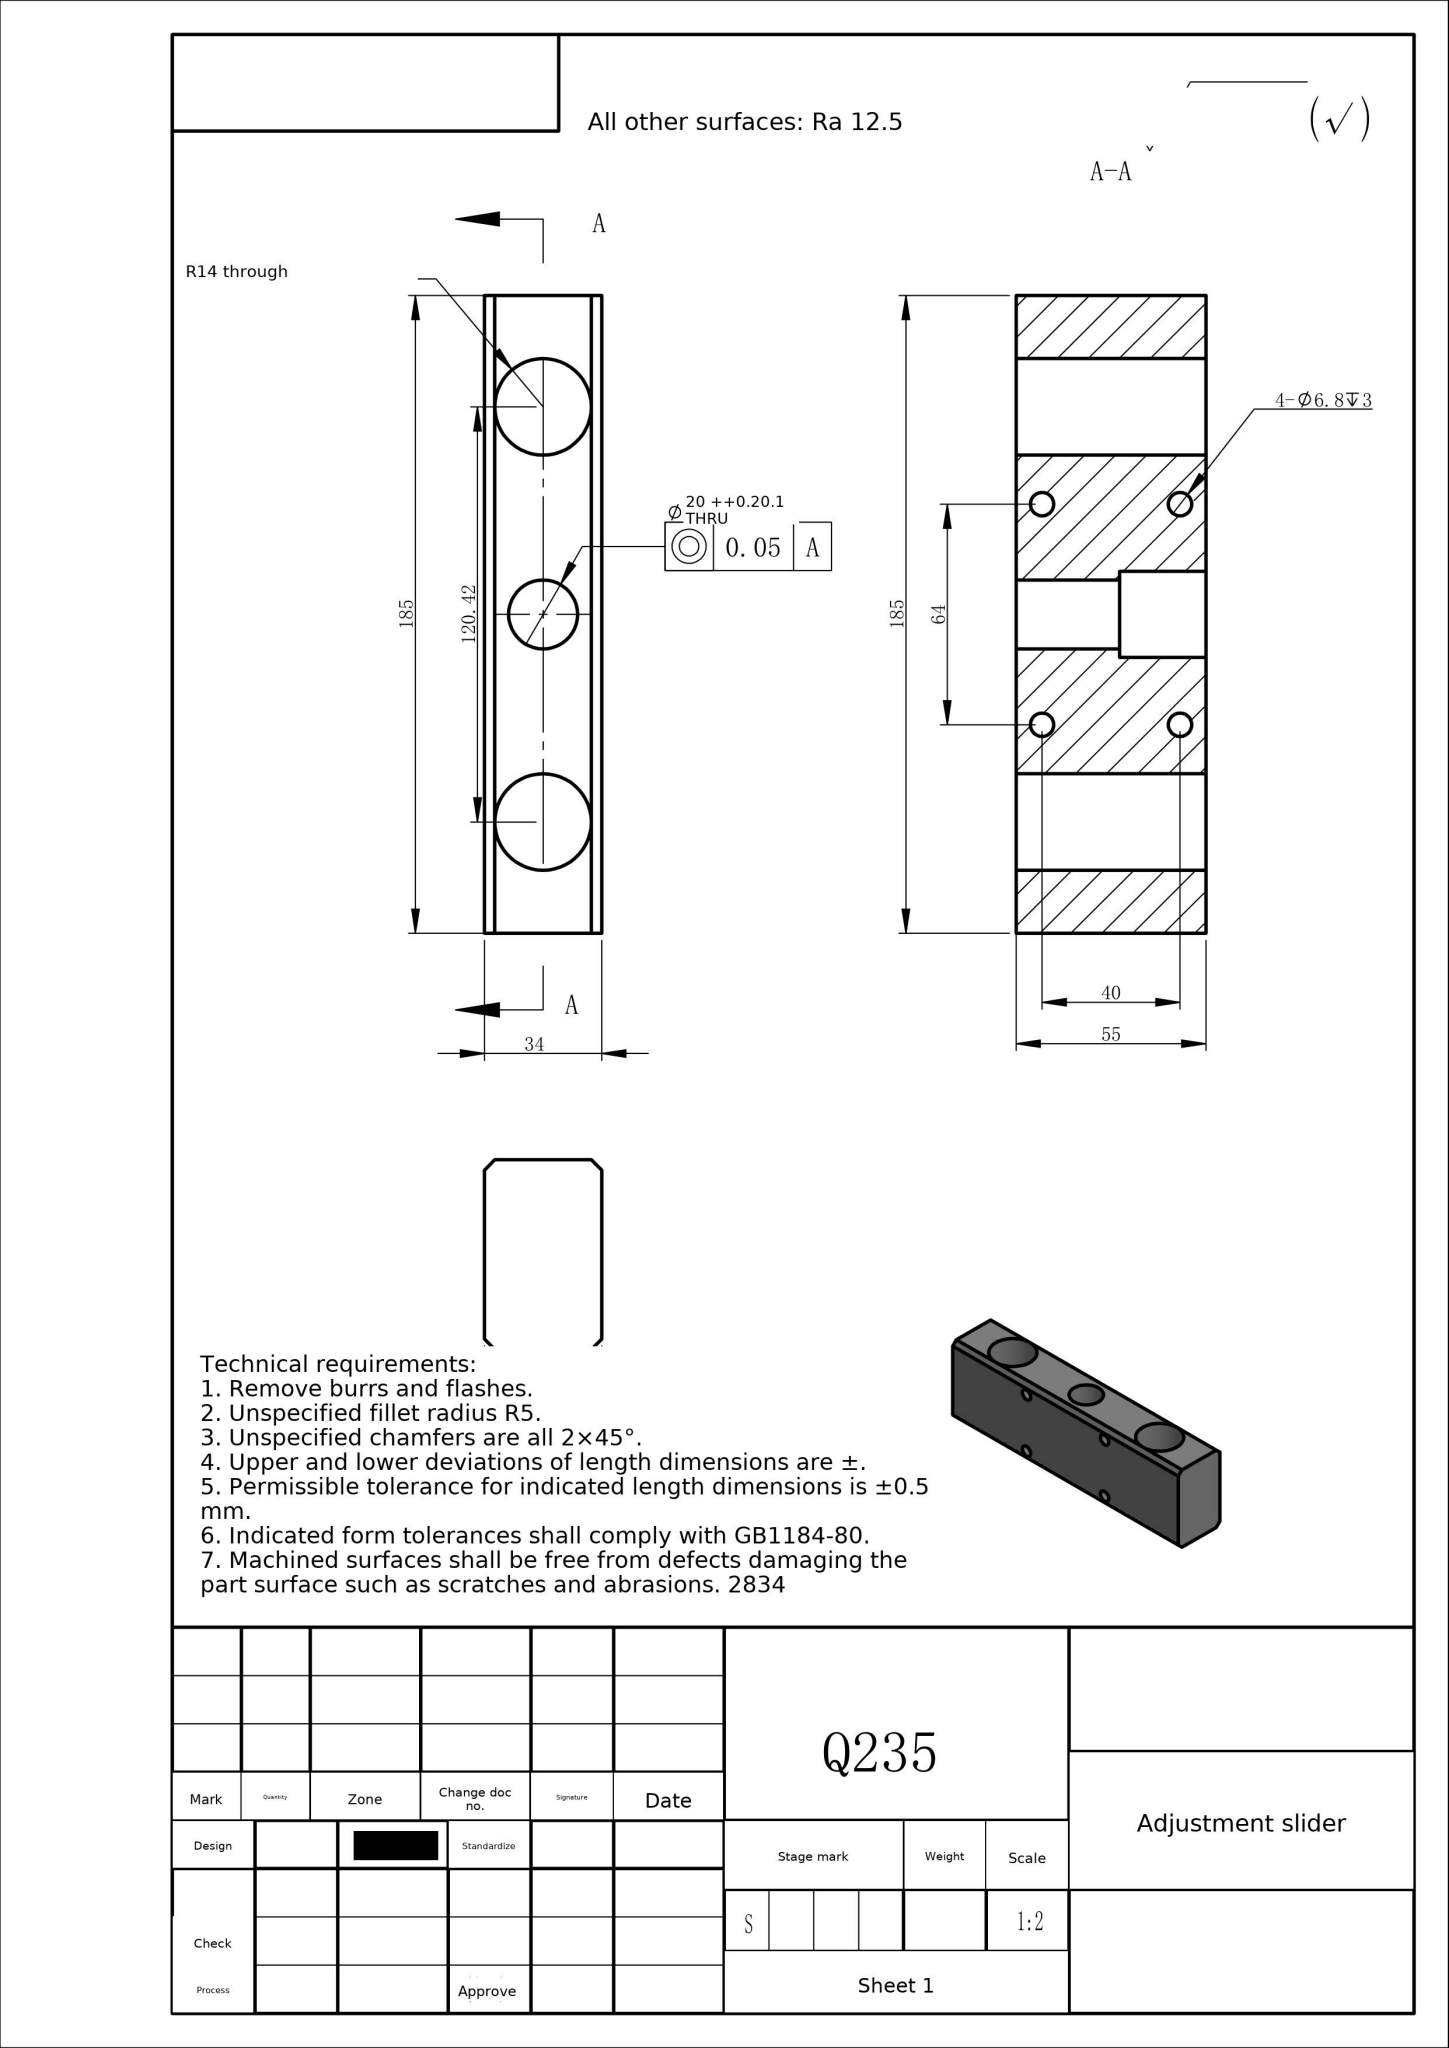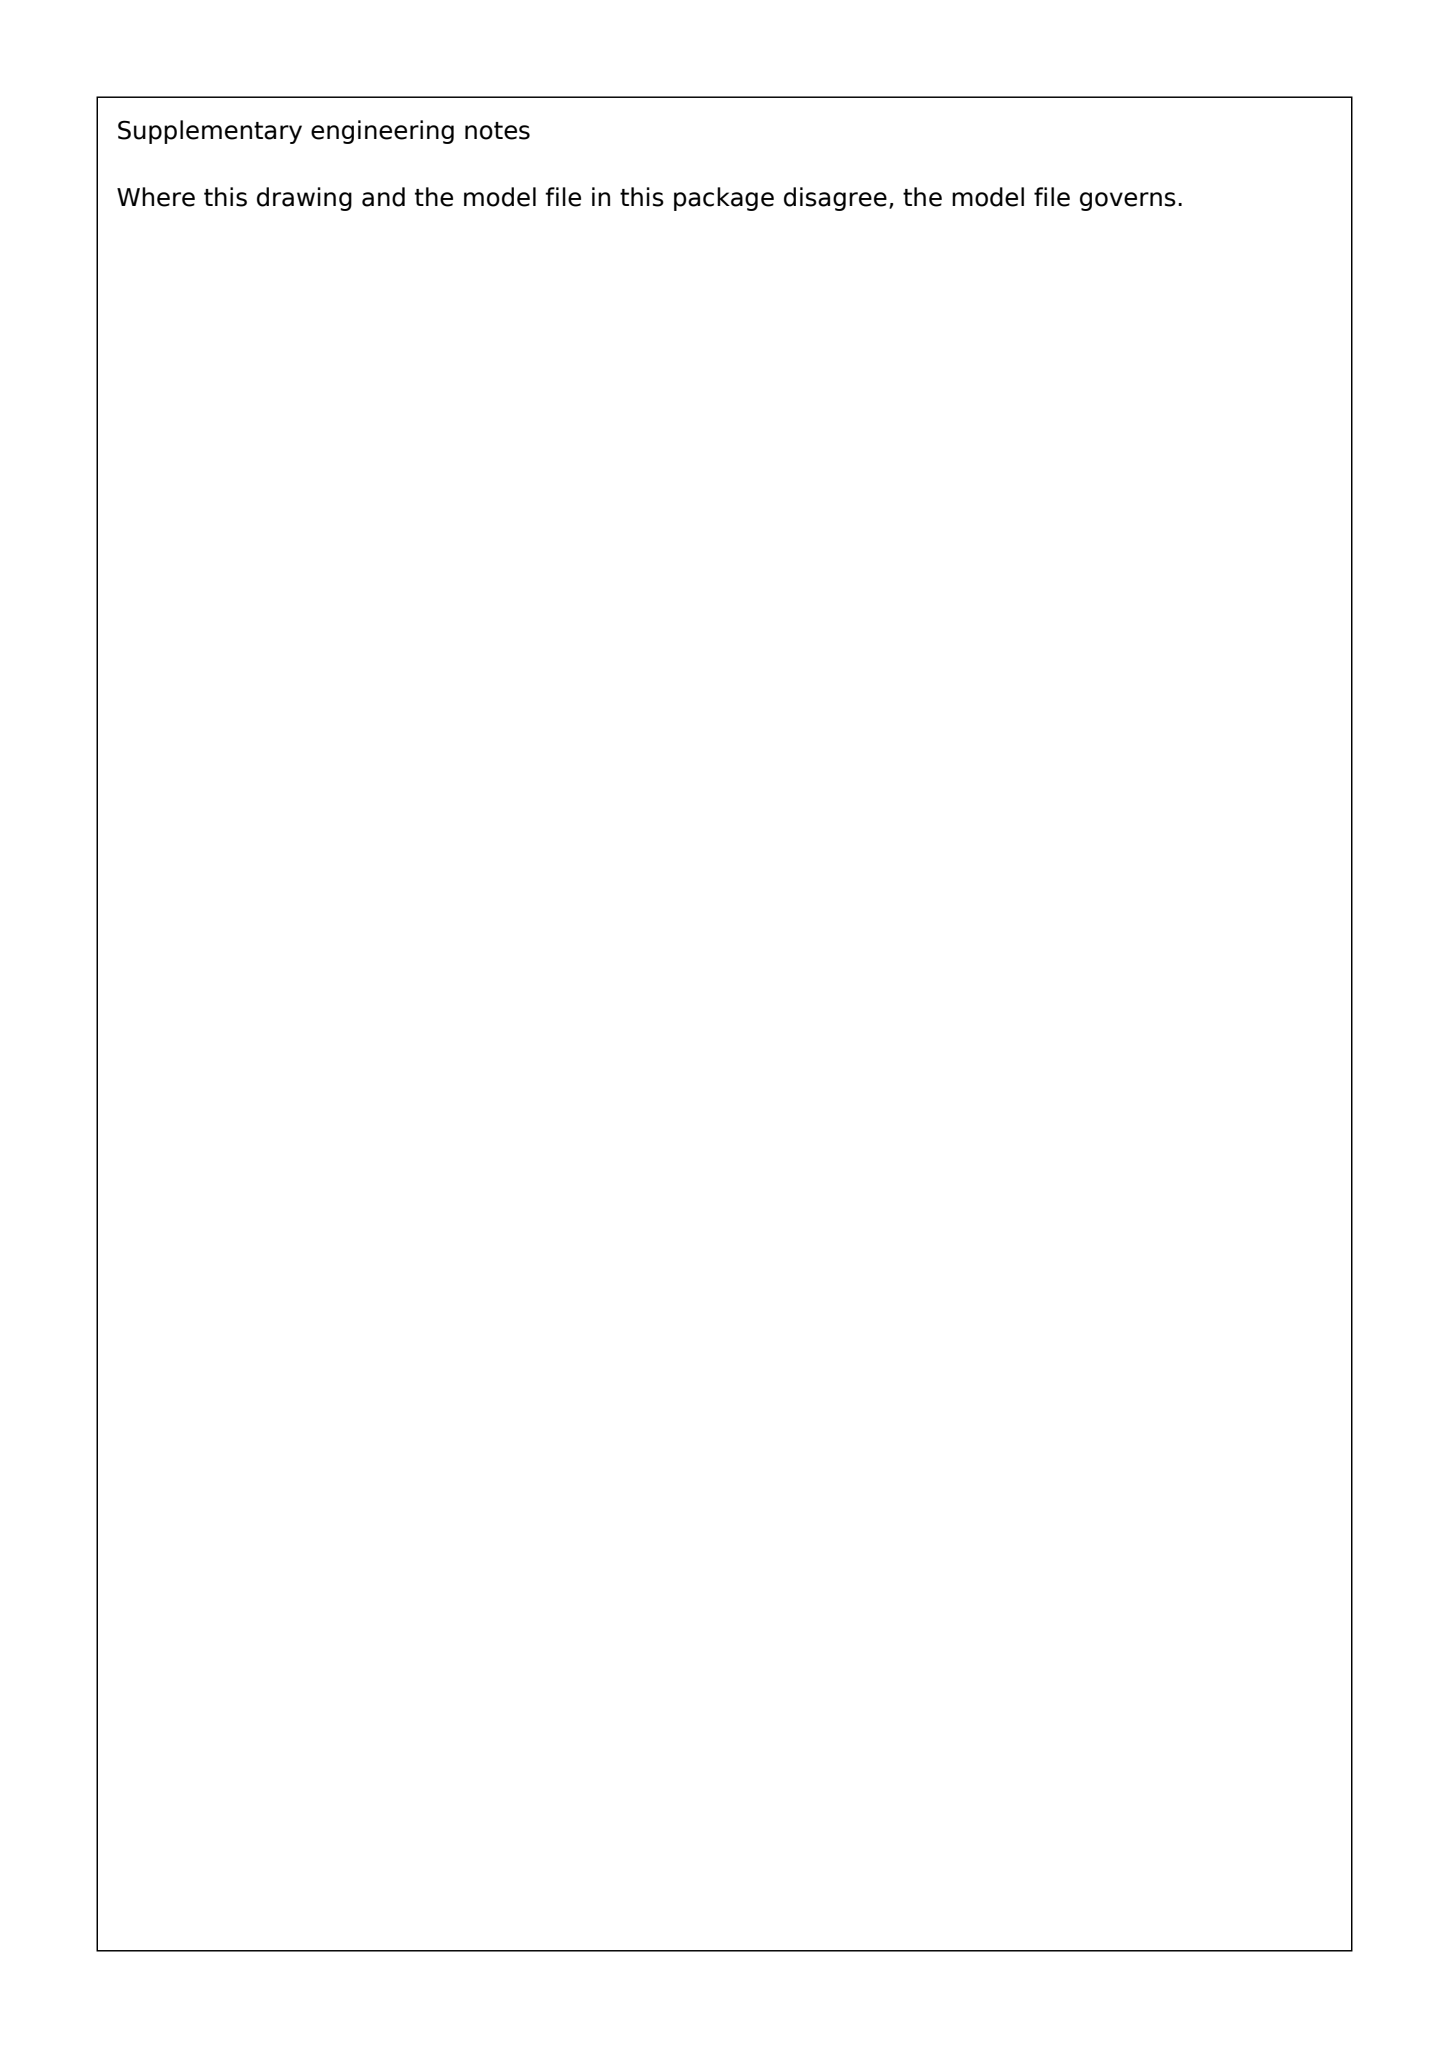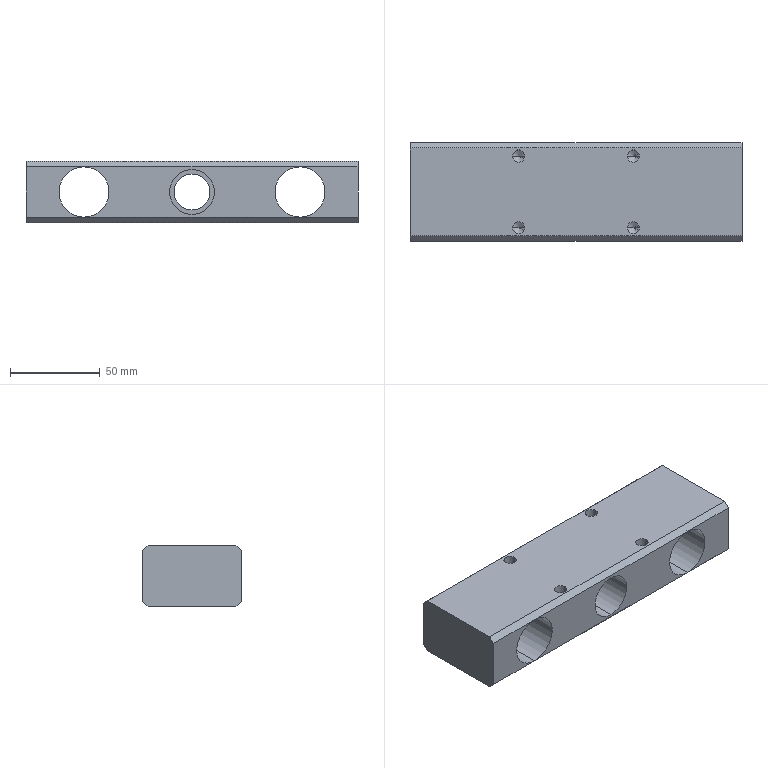Part | SolidWorks | drawing in inches | material Q235 | 1 solid | 39 faces | box 185 x 55 x 34 mm | volume 250186 mm3 | cylinder 16 | plane 15 | cone 8 | commonest cylinder face diameters 6.8 x8 28 x4 25 x2 20 x2